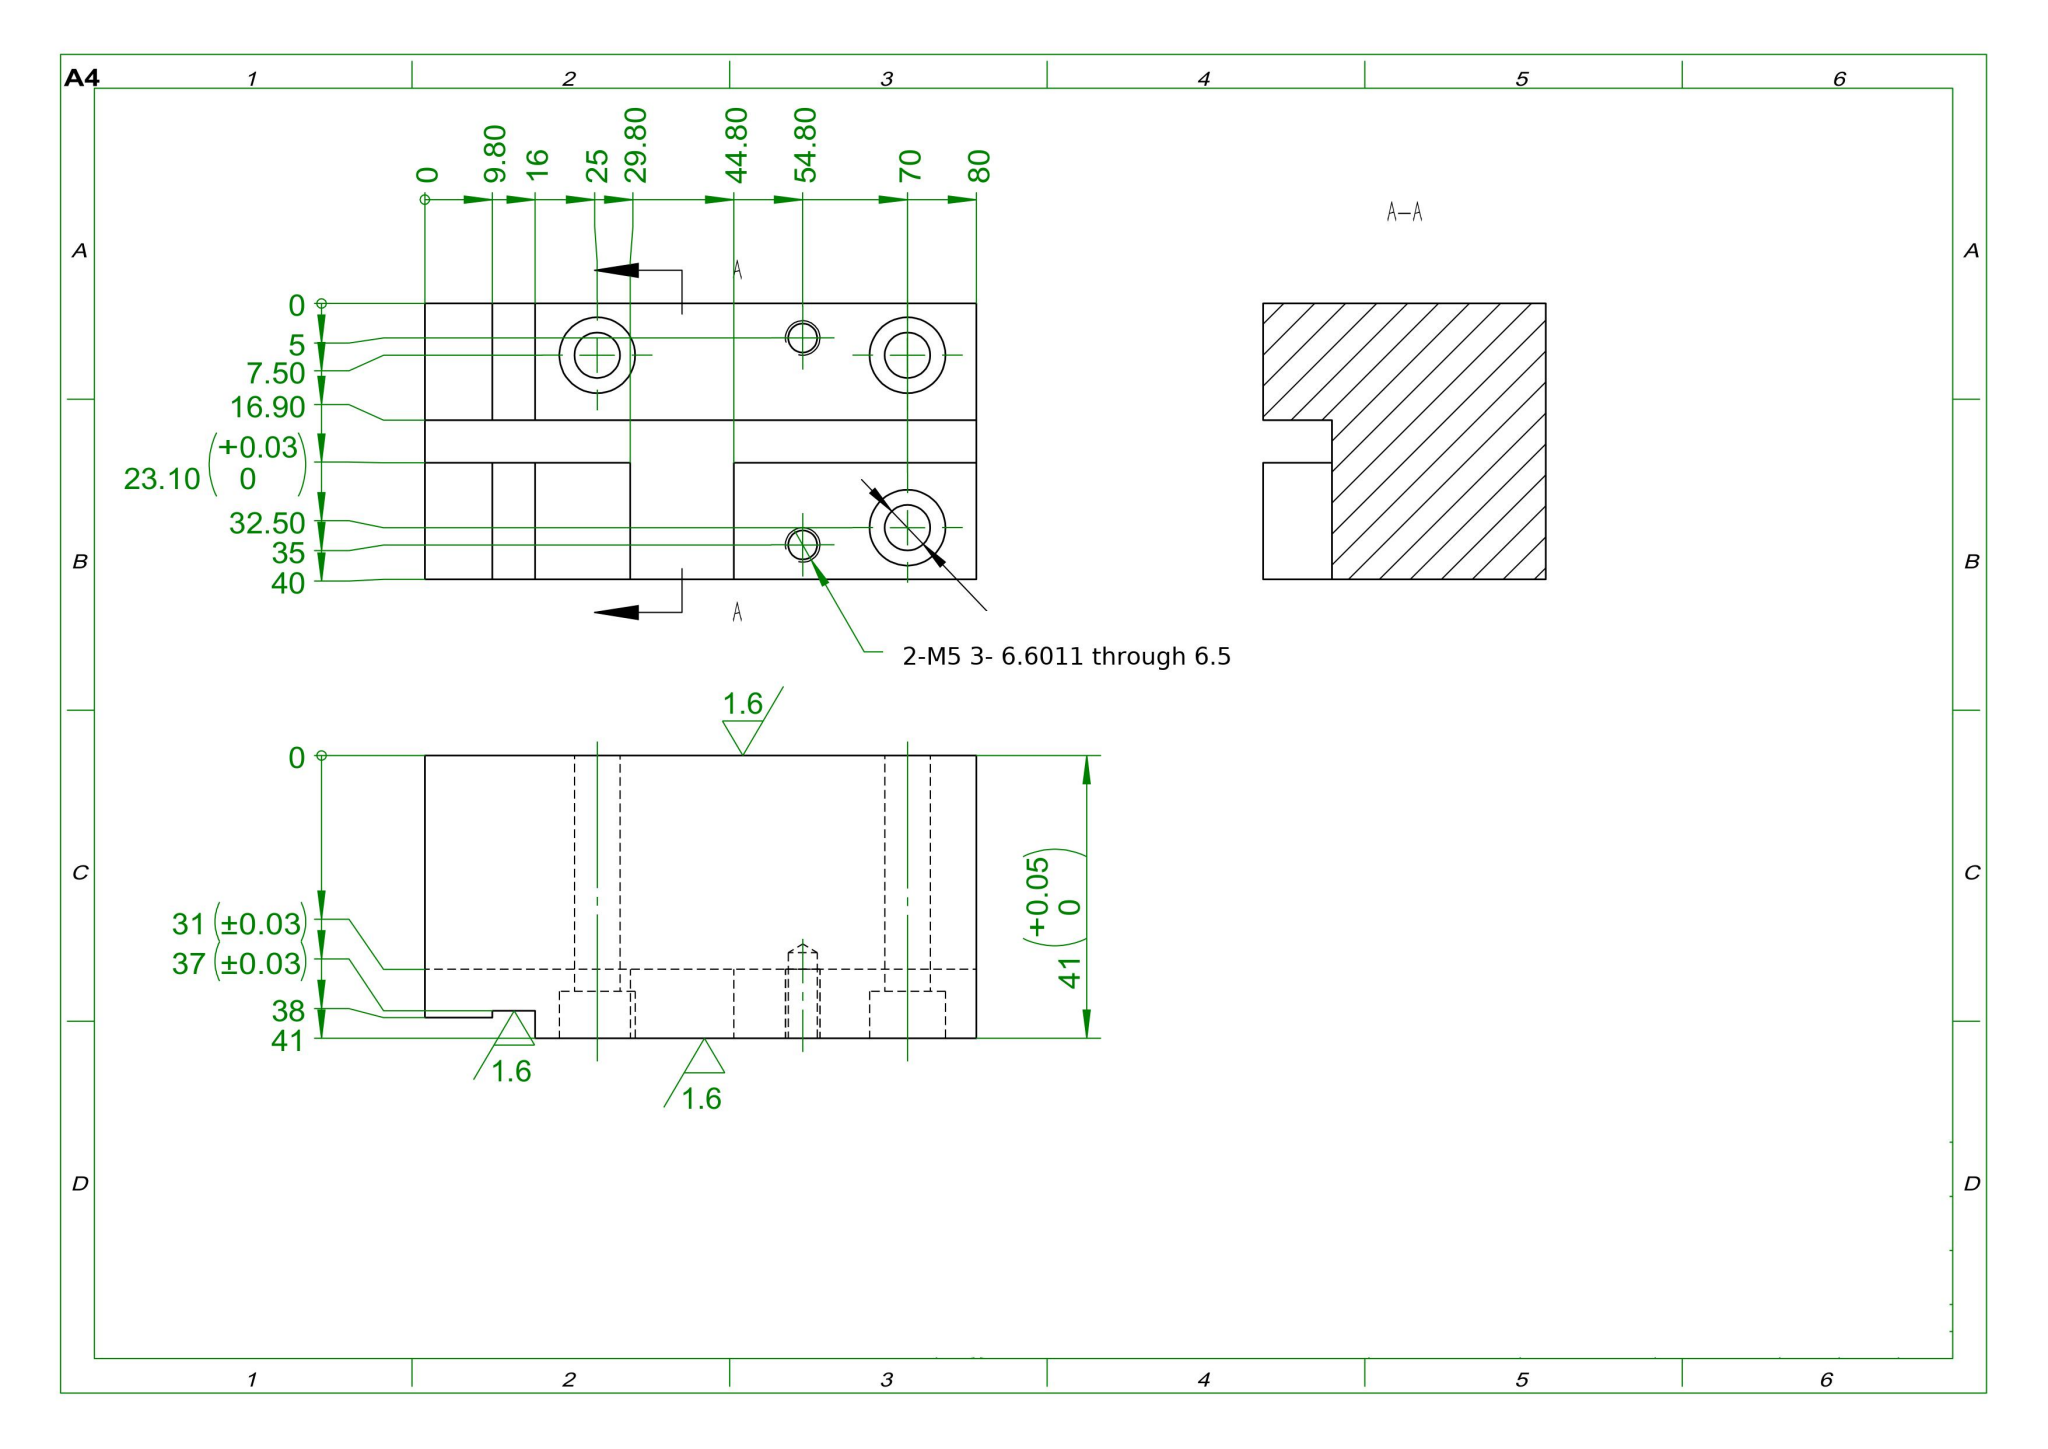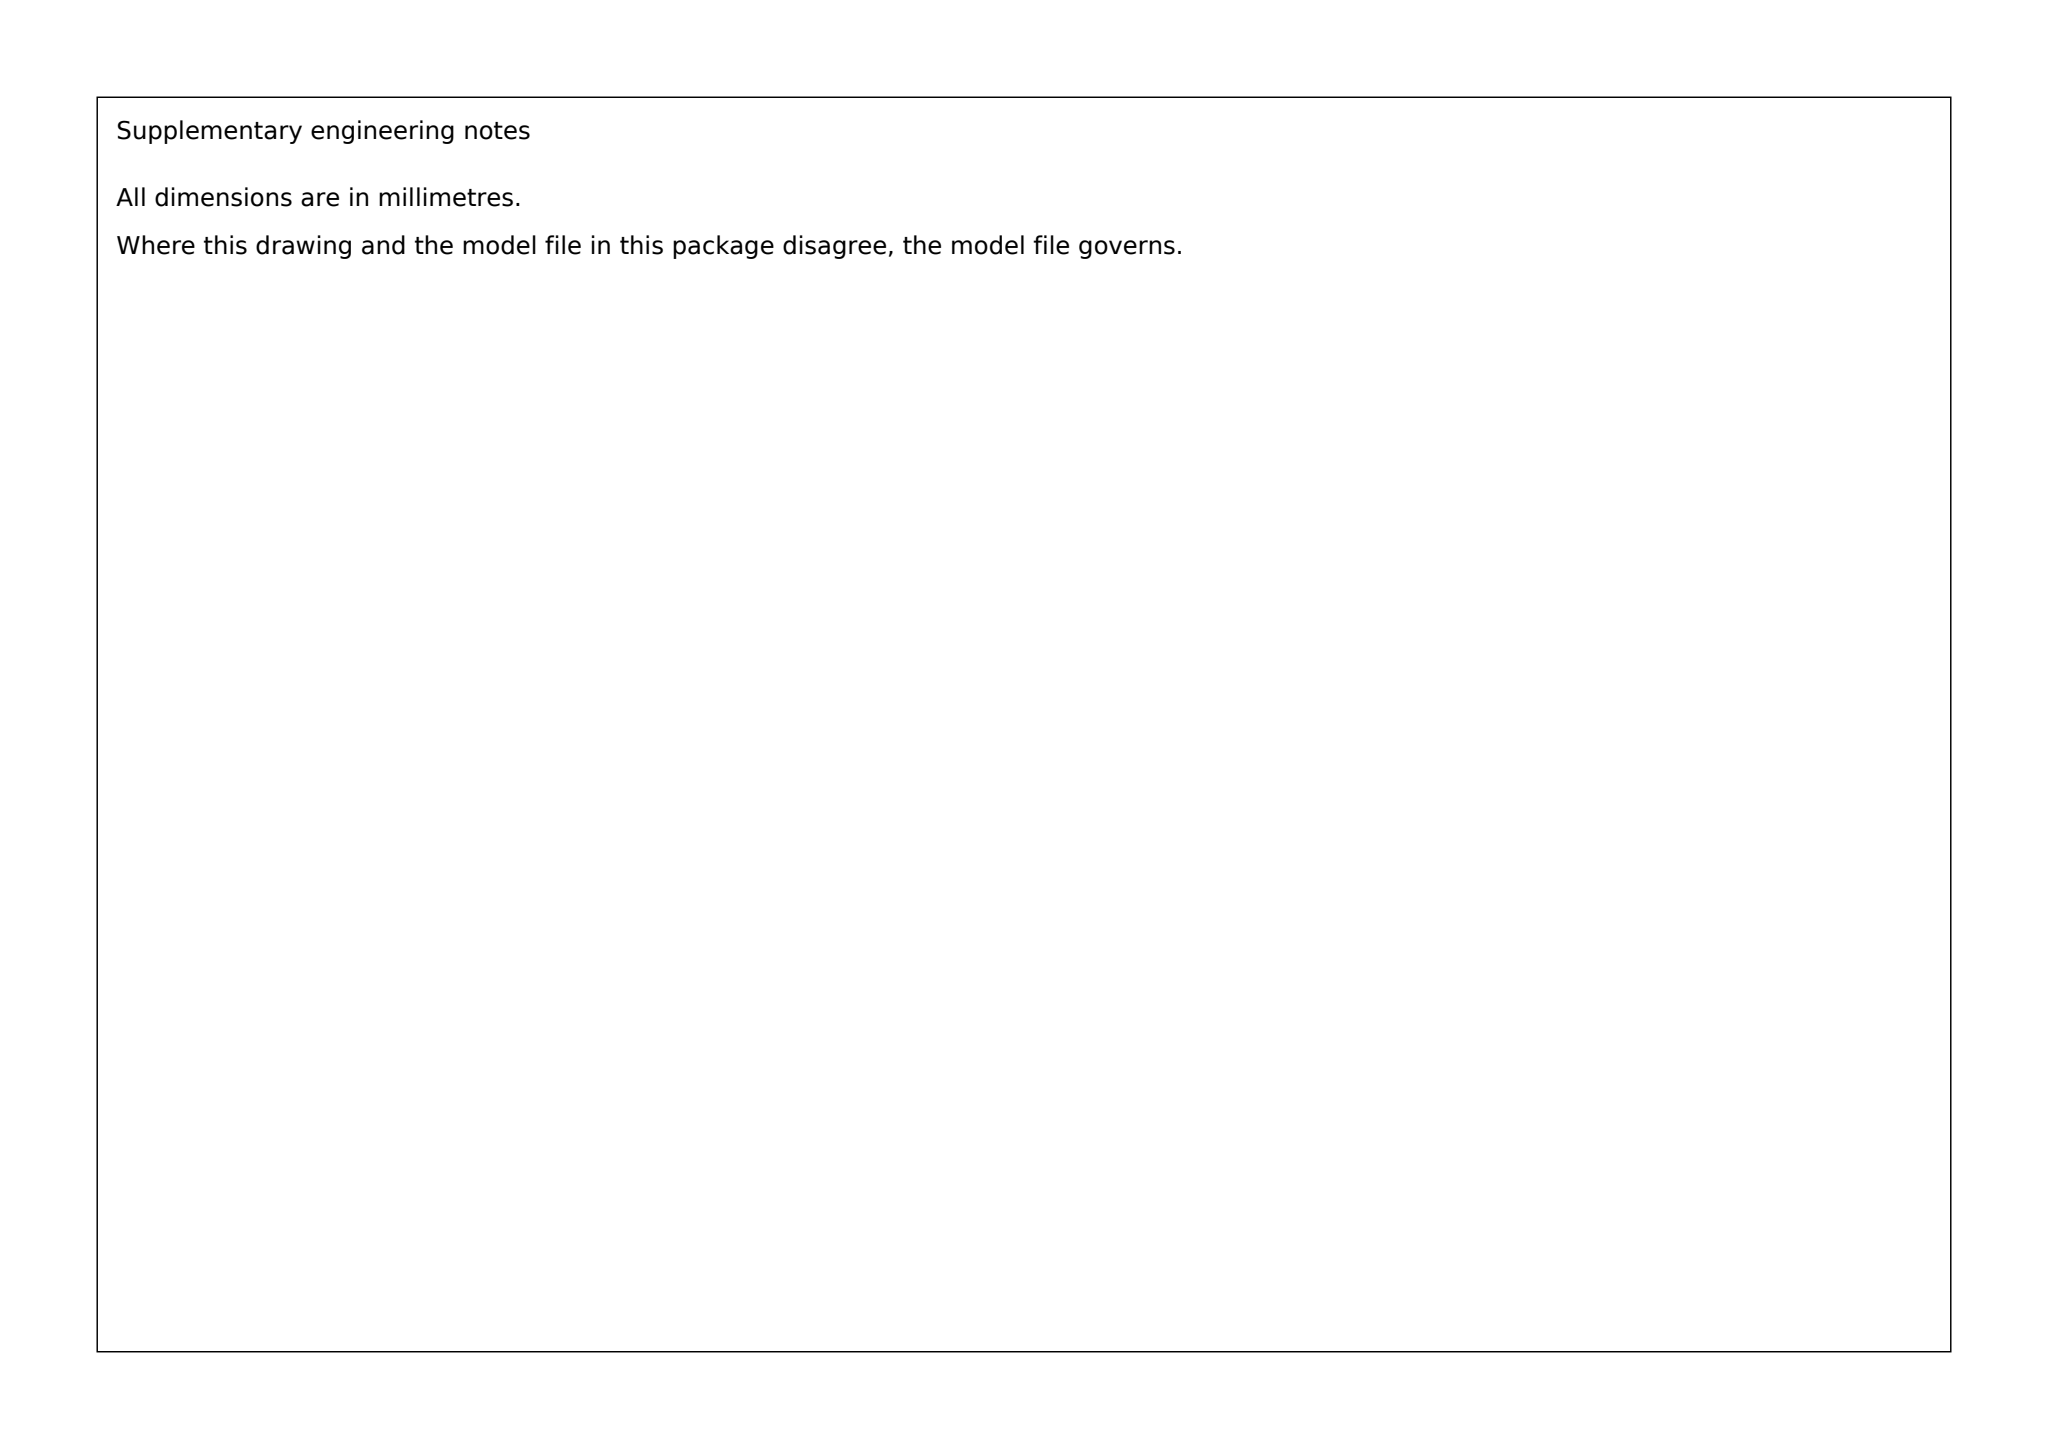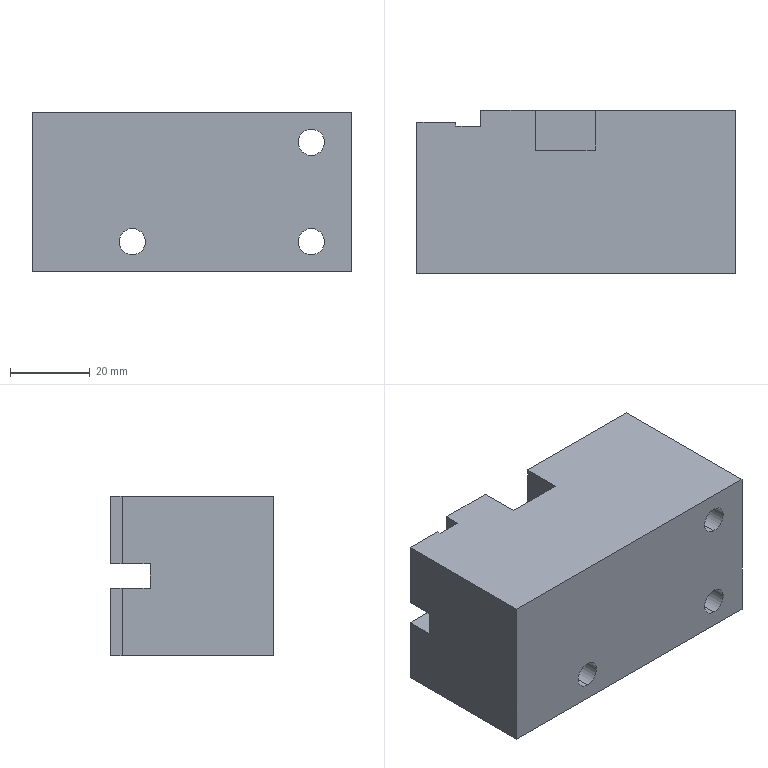Part | SolidWorks | mm | 1 solid | 45 faces | box 80 x 41 x 40 mm | volume 116069 mm3 | plane 25 | cylinder 16 | cone 4 | commonest cylinder face diameters 11 x6 6.6 x6 4.2 x4
build123d program:
from build123d import *

# Parameters (mm, degrees)
BOSS_EXTRUDE1_DEPTH                               = 40
SKETCH2_W                                         = 6.2
SKETCH2_H                                         = 20
CUT_EXTRUDE1_DEPTH                                = 100
SKETCH3_W                                         = 15
SKETCH3_H                                         = 16.9
CUT_EXTRUDE2_DEPTH                                = 10
HOLE_SIZE_ACCORDING_TO_TYPE_1_OF_HEXA_D           = 6.6
HOLE_SIZE_ACCORDING_TO_TYPE_1_OF_HEXA_CBORE_D     = 11
HOLE_SIZE_ACCORDING_TO_TYPE_1_OF_HEXA_CBORE_DEPTH = 6.8
M5_TAPPED_HOLE1_D                                 = 4.2
M5_TAPPED_HOLE1_DEPTH                             = 12.4
M5_TAPPED_HOLE1_TIP                               = 1.262


with BuildPart() as part:
    # Sketch1 → Boss-Extrude1 (new body)
    with BuildSketch(Plane.XY):
        Polygon((0, 0), (9.8, 0), (9.8, -1), (16, -1), (16, 3), (80, 3), (80, -38), (0, -38), align=None)
    extrude(amount=BOSS_EXTRUDE1_DEPTH)

    # Sketch2 → Cut-Extrude1 (cut)
    with BuildSketch(Plane.ZY):
        with Locations((20, 3)):
            Rectangle(SKETCH2_W, SKETCH2_H)
    extrude(amount=-CUT_EXTRUDE1_DEPTH, mode=Mode.SUBTRACT)

    # Sketch3 → Cut-Extrude2 (cut)
    with BuildSketch(Plane(origin=(0, 3, 0), x_dir=(1, 0, 0), z_dir=(0, 1, 0))):
        with Locations((37.3, -31.55)):
            Rectangle(SKETCH3_W, SKETCH3_H)
    extrude(amount=-CUT_EXTRUDE2_DEPTH, mode=Mode.SUBTRACT)

    # Hole Size _ according to_ Type 1 of Hexa (through all)
    with Locations(Plane(origin=(0, 3, 0), x_dir=(1, 0, 0), z_dir=(0, 1, 0))):
        with Locations((25, -7.5), (70, -7.5), (70, -32.5)):
            CounterBoreHole(HOLE_SIZE_ACCORDING_TO_TYPE_1_OF_HEXA_D / 2, HOLE_SIZE_ACCORDING_TO_TYPE_1_OF_HEXA_CBORE_D / 2, HOLE_SIZE_ACCORDING_TO_TYPE_1_OF_HEXA_CBORE_DEPTH)

    # M5 Tapped Hole1
    with Locations(Plane(origin=(0, 3, 0), x_dir=(1, 0, 0), z_dir=(0, 1, 0))):
        with Locations((54.8, -5), (54.8, -35)):
            Hole(M5_TAPPED_HOLE1_D / 2, depth=M5_TAPPED_HOLE1_DEPTH)
            with Locations((0, 0, -(M5_TAPPED_HOLE1_DEPTH + M5_TAPPED_HOLE1_TIP / 2))):  # 118° drill point
                Cone(0, M5_TAPPED_HOLE1_D / 2, M5_TAPPED_HOLE1_TIP, mode=Mode.SUBTRACT)


solid = part.part